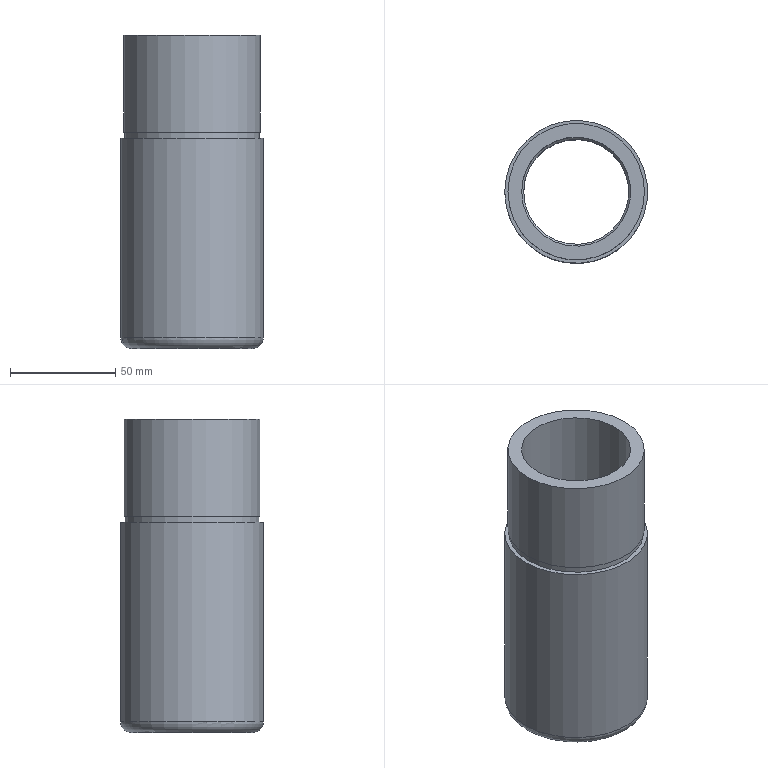Component | NX | OUTER_GUIDE_BUSH | 1 solid | 17 faces | box 68 x 68 x 149 mm | volume 223119 mm3 | cylinder 8 | plane 4 | torus 4 | cone 1 | commonest cylinder face diameters 50 x4 64 x1 68 x1 51.928 x1 64.974 x1
STEP:
#1=CARTESIAN_POINT('',(0.,0.,0.));
#2=DIRECTION('',(0.,0.,1.));
#3=DIRECTION('',(1.,0.,0.));
#4=AXIS2_PLACEMENT_3D('',#1,#2,#3);
#5=CARTESIAN_POINT('',(-322.,-290.,198.));
#6=VERTEX_POINT('',#5);
#7=CARTESIAN_POINT('',(-290.,-290.,198.));
#8=DIRECTION('',(0.,0.,-1.));
#9=DIRECTION('',(-1.,0.0000016,0.));
#10=AXIS2_PLACEMENT_3D('',#7,#8,#9);
#11=CIRCLE('',#10,32.);
#12=CARTESIAN_POINT('',(-257.513,-290.,198.));
#13=DIRECTION('',(0.,0.,1.));
#14=DIRECTION('',(1.,-0.0000016,0.));
#15=AXIS2_PLACEMENT_3D('',#12,#13,#14);
#16=PLANE('',#15);
#17=CARTESIAN_POINT('',(-64.487,-0.));
#18=CARTESIAN_POINT('',(-64.487,55.426));
#19=CARTESIAN_POINT('',(-16.487,27.713));
#20=CARTESIAN_POINT('',(31.513,0.));
#21=CARTESIAN_POINT('',(-16.487,-27.713));
#22=CARTESIAN_POINT('',(-64.487,-55.426));
#23=CARTESIAN_POINT('',(-64.487,-0.));
#24=(BOUNDED_CURVE()B_SPLINE_CURVE(2,(#17,#18,#19,#20,#21,#22,#23),.UNSPECIFIED.,.T.,.F.)B_SPLINE_CURVE_WITH_KNOTS((1,2,2,2,2,1),(-2.094,0.,2.094,4.189,6.283,8.378),.UNSPECIFIED.)CURVE()GEOMETRIC_REPRESENTATION_ITEM()RATIONAL_B_SPLINE_CURVE((1.,0.5,1.,0.5,1.,0.5,1.))REPRESENTATION_ITEM(''));
#25=(GEOMETRIC_REPRESENTATION_CONTEXT(2)PARAMETRIC_REPRESENTATION_CONTEXT()REPRESENTATION_CONTEXT('',''));
#26=DEFINITIONAL_REPRESENTATION('',(#24),#25);
#27=PCURVE('',#16,#26);
#28=CARTESIAN_POINT('',(-290.,-290.,95.));
#29=DIRECTION('',(0.,0.,-1.));
#30=DIRECTION('',(-1.,0.0000016,0.));
#31=AXIS2_PLACEMENT_3D('',#28,#29,#30);
#32=CYLINDRICAL_SURFACE('',#31,32.);
#33=CARTESIAN_POINT('',(0.,-103.));
#34=DIRECTION('',(1.,0.));
#35=VECTOR('',#34,1.);
#36=LINE('',#33,#35);
#37=(GEOMETRIC_REPRESENTATION_CONTEXT(2)PARAMETRIC_REPRESENTATION_CONTEXT()REPRESENTATION_CONTEXT('',''));
#38=DEFINITIONAL_REPRESENTATION('',(#36),#37);
#39=PCURVE('',#32,#38);
#40=SURFACE_CURVE('',#11,(#27,#39),.PCURVE_S1.);
#41=EDGE_CURVE('',#6,#6,#40,.T.);
#42=ORIENTED_EDGE('',*,*,#41,.F.);
#43=EDGE_LOOP('',(#42));
#44=FACE_BOUND('',#43,.T.);
#45=CARTESIAN_POINT('',(-322.487,-290.,198.));
#46=VERTEX_POINT('',#45);
#47=CARTESIAN_POINT('',(-290.,-290.,198.));
#48=DIRECTION('',(0.,0.,-1.));
#49=DIRECTION('',(-1.,0.0000016,0.));
#50=AXIS2_PLACEMENT_3D('',#47,#48,#49);
#51=CIRCLE('',#50,32.487);
#52=CARTESIAN_POINT('',(-64.974,-0.));
#53=CARTESIAN_POINT('',(-64.974,56.269));
#54=CARTESIAN_POINT('',(-16.243,28.134));
#55=CARTESIAN_POINT('',(32.487,0.));
#56=CARTESIAN_POINT('',(-16.243,-28.134));
#57=CARTESIAN_POINT('',(-64.974,-56.269));
#58=CARTESIAN_POINT('',(-64.974,-0.));
#59=(BOUNDED_CURVE()B_SPLINE_CURVE(2,(#52,#53,#54,#55,#56,#57,#58),.UNSPECIFIED.,.T.,.F.)B_SPLINE_CURVE_WITH_KNOTS((1,2,2,2,2,1),(-2.094,0.,2.094,4.189,6.283,8.378),.UNSPECIFIED.)CURVE()GEOMETRIC_REPRESENTATION_ITEM()RATIONAL_B_SPLINE_CURVE((1.,0.5,1.,0.5,1.,0.5,1.))REPRESENTATION_ITEM(''));
#60=(GEOMETRIC_REPRESENTATION_CONTEXT(2)PARAMETRIC_REPRESENTATION_CONTEXT()REPRESENTATION_CONTEXT('',''));
#61=DEFINITIONAL_REPRESENTATION('',(#59),#60);
#62=PCURVE('',#16,#61);
#63=CARTESIAN_POINT('',(-290.,-290.,95.));
#64=DIRECTION('',(0.,0.,-1.));
#65=DIRECTION('',(-1.,0.0000016,0.));
#66=AXIS2_PLACEMENT_3D('',#63,#64,#65);
#67=CYLINDRICAL_SURFACE('',#66,32.487);
#68=CARTESIAN_POINT('',(0.,-103.));
#69=DIRECTION('',(1.,0.));
#70=VECTOR('',#69,1.);
#71=LINE('',#68,#70);
#72=(GEOMETRIC_REPRESENTATION_CONTEXT(2)PARAMETRIC_REPRESENTATION_CONTEXT()REPRESENTATION_CONTEXT('',''));
#73=DEFINITIONAL_REPRESENTATION('',(#71),#72);
#74=PCURVE('',#67,#73);
#75=SURFACE_CURVE('',#51,(#62,#74),.PCURVE_S1.);
#76=EDGE_CURVE('',#46,#46,#75,.T.);
#77=ORIENTED_EDGE('',*,*,#76,.T.);
#78=EDGE_LOOP('',(#77));
#79=FACE_BOUND('',#78,.T.);
#80=ADVANCED_FACE('',(#44,#79),#16,.F.);
#81=CARTESIAN_POINT('',(-322.,-290.,195.));
#82=VERTEX_POINT('',#81);
#83=CARTESIAN_POINT('',(-290.,-290.,195.));
#84=DIRECTION('',(0.,0.,-1.));
#85=DIRECTION('',(-1.,0.0000016,0.));
#86=AXIS2_PLACEMENT_3D('',#83,#84,#85);
#87=CIRCLE('',#86,32.);
#88=CARTESIAN_POINT('',(0.,-100.));
#89=DIRECTION('',(1.,0.));
#90=VECTOR('',#89,1.);
#91=LINE('',#88,#90);
#92=(GEOMETRIC_REPRESENTATION_CONTEXT(2)PARAMETRIC_REPRESENTATION_CONTEXT()REPRESENTATION_CONTEXT('',''));
#93=DEFINITIONAL_REPRESENTATION('',(#91),#92);
#94=PCURVE('',#32,#93);
#95=CARTESIAN_POINT('',(-258.,-290.,195.));
#96=DIRECTION('',(0.,0.,-1.));
#97=DIRECTION('',(-1.,0.0000016,0.));
#98=AXIS2_PLACEMENT_3D('',#95,#96,#97);
#99=PLANE('',#98);
#100=CARTESIAN_POINT('',(32.,-0.));
#101=DIRECTION('',(1.,-0.));
#102=AXIS2_PLACEMENT_2D('',#100,#101);
#103=CIRCLE('',#102,32.);
#104=(GEOMETRIC_REPRESENTATION_CONTEXT(2)PARAMETRIC_REPRESENTATION_CONTEXT()REPRESENTATION_CONTEXT('',''));
#105=DEFINITIONAL_REPRESENTATION('',(#103),#104);
#106=PCURVE('',#99,#105);
#107=SURFACE_CURVE('',#87,(#94,#106),.PCURVE_S1.);
#108=EDGE_CURVE('',#82,#82,#107,.T.);
#109=ORIENTED_EDGE('',*,*,#108,.F.);
#110=CARTESIAN_POINT('',(-322.,-290.,198.));
#111=CARTESIAN_POINT('',(-322.,-290.,195.));
#112=B_SPLINE_CURVE_WITH_KNOTS('',1,(#110,#111),.UNSPECIFIED.,.F.,.F.,(2,2),(-103.,-100.),.PIECEWISE_BEZIER_KNOTS.);
#113=CARTESIAN_POINT('',(0.,0.));
#114=DIRECTION('',(0.,1.));
#115=VECTOR('',#114,1.);
#116=LINE('',#113,#115);
#117=(GEOMETRIC_REPRESENTATION_CONTEXT(2)PARAMETRIC_REPRESENTATION_CONTEXT()REPRESENTATION_CONTEXT('',''));
#118=DEFINITIONAL_REPRESENTATION('',(#116),#117);
#119=PCURVE('',#32,#118);
#120=CARTESIAN_POINT('',(6.283,0.));
#121=DIRECTION('',(0.,1.));
#122=VECTOR('',#121,1.);
#123=LINE('',#120,#122);
#124=(GEOMETRIC_REPRESENTATION_CONTEXT(2)PARAMETRIC_REPRESENTATION_CONTEXT()REPRESENTATION_CONTEXT('',''));
#125=DEFINITIONAL_REPRESENTATION('',(#123),#124);
#126=PCURVE('',#32,#125);
#127=SEAM_CURVE('',#112,(#119,#126),.PCURVE_S1.);
#128=EDGE_CURVE('',#6,#82,#127,.T.);
#129=ORIENTED_EDGE('',*,*,#128,.F.);
#130=ORIENTED_EDGE('',*,*,#41,.T.);
#131=ORIENTED_EDGE('',*,*,#128,.T.);
#132=EDGE_LOOP('',(#109,#129,#130,#131));
#133=FACE_BOUND('',#132,.T.);
#134=ADVANCED_FACE('',(#133),#32,.T.);
#135=CARTESIAN_POINT('',(-324.,-290.,195.));
#136=VERTEX_POINT('',#135);
#137=CARTESIAN_POINT('',(-290.,-290.,195.));
#138=DIRECTION('',(0.,0.,-1.));
#139=DIRECTION('',(-1.,0.0000016,0.));
#140=AXIS2_PLACEMENT_3D('',#137,#138,#139);
#141=CIRCLE('',#140,34.);
#142=CARTESIAN_POINT('',(32.,-0.));
#143=DIRECTION('',(1.,-0.));
#144=AXIS2_PLACEMENT_2D('',#142,#143);
#145=CIRCLE('',#144,34.);
#146=(GEOMETRIC_REPRESENTATION_CONTEXT(2)PARAMETRIC_REPRESENTATION_CONTEXT()REPRESENTATION_CONTEXT('',''));
#147=DEFINITIONAL_REPRESENTATION('',(#145),#146);
#148=PCURVE('',#99,#147);
#149=CARTESIAN_POINT('',(-290.,-290.,95.));
#150=DIRECTION('',(0.,0.,-1.));
#151=DIRECTION('',(-1.,0.0000016,0.));
#152=AXIS2_PLACEMENT_3D('',#149,#150,#151);
#153=CYLINDRICAL_SURFACE('',#152,34.);
#154=CARTESIAN_POINT('',(0.,-100.));
#155=DIRECTION('',(1.,0.));
#156=VECTOR('',#155,1.);
#157=LINE('',#154,#156);
#158=(GEOMETRIC_REPRESENTATION_CONTEXT(2)PARAMETRIC_REPRESENTATION_CONTEXT()REPRESENTATION_CONTEXT('',''));
#159=DEFINITIONAL_REPRESENTATION('',(#157),#158);
#160=PCURVE('',#153,#159);
#161=SURFACE_CURVE('',#141,(#148,#160),.PCURVE_S1.);
#162=EDGE_CURVE('',#136,#136,#161,.T.);
#163=ORIENTED_EDGE('',*,*,#162,.F.);
#164=EDGE_LOOP('',(#163));
#165=FACE_BOUND('',#164,.T.);
#166=ORIENTED_EDGE('',*,*,#108,.T.);
#167=EDGE_LOOP('',(#166));
#168=FACE_BOUND('',#167,.T.);
#169=ADVANCED_FACE('',(#165,#168),#99,.F.);
#170=CARTESIAN_POINT('',(-324.,-290.,100.));
#171=VERTEX_POINT('',#170);
#172=CARTESIAN_POINT('',(-290.,-290.,100.));
#173=DIRECTION('',(0.,0.,-1.));
#174=DIRECTION('',(-1.,0.0000016,0.));
#175=AXIS2_PLACEMENT_3D('',#172,#173,#174);
#176=CIRCLE('',#175,34.);
#177=CARTESIAN_POINT('',(0.,-5.));
#178=DIRECTION('',(1.,0.));
#179=VECTOR('',#178,1.);
#180=LINE('',#177,#179);
#181=(GEOMETRIC_REPRESENTATION_CONTEXT(2)PARAMETRIC_REPRESENTATION_CONTEXT()REPRESENTATION_CONTEXT('',''));
#182=DEFINITIONAL_REPRESENTATION('',(#180),#181);
#183=PCURVE('',#153,#182);
#184=CARTESIAN_POINT('',(-290.,-290.,100.));
#185=DIRECTION('',(0.,0.,-1.));
#186=DIRECTION('',(-1.,0.0000016,0.));
#187=AXIS2_PLACEMENT_3D('',#184,#185,#186);
#188=TOROIDAL_SURFACE('',#187,29.,5.);
#189=CARTESIAN_POINT('',(0.,6.283));
#190=DIRECTION('',(1.,0.));
#191=VECTOR('',#190,1.);
#192=LINE('',#189,#191);
#193=(GEOMETRIC_REPRESENTATION_CONTEXT(2)PARAMETRIC_REPRESENTATION_CONTEXT()REPRESENTATION_CONTEXT('',''));
#194=DEFINITIONAL_REPRESENTATION('',(#192),#193);
#195=PCURVE('',#188,#194);
#196=SURFACE_CURVE('',#176,(#183,#195),.PCURVE_S1.);
#197=EDGE_CURVE('',#171,#171,#196,.T.);
#198=ORIENTED_EDGE('',*,*,#197,.F.);
#199=CARTESIAN_POINT('',(-324.,-290.,195.));
#200=CARTESIAN_POINT('',(-324.,-290.,100.));
#201=B_SPLINE_CURVE_WITH_KNOTS('',1,(#199,#200),.UNSPECIFIED.,.F.,.F.,(2,2),(-100.,-5.),.PIECEWISE_BEZIER_KNOTS.);
#202=CARTESIAN_POINT('',(0.,0.));
#203=DIRECTION('',(0.,1.));
#204=VECTOR('',#203,1.);
#205=LINE('',#202,#204);
#206=(GEOMETRIC_REPRESENTATION_CONTEXT(2)PARAMETRIC_REPRESENTATION_CONTEXT()REPRESENTATION_CONTEXT('',''));
#207=DEFINITIONAL_REPRESENTATION('',(#205),#206);
#208=PCURVE('',#153,#207);
#209=CARTESIAN_POINT('',(6.283,0.));
#210=DIRECTION('',(0.,1.));
#211=VECTOR('',#210,1.);
#212=LINE('',#209,#211);
#213=(GEOMETRIC_REPRESENTATION_CONTEXT(2)PARAMETRIC_REPRESENTATION_CONTEXT()REPRESENTATION_CONTEXT('',''));
#214=DEFINITIONAL_REPRESENTATION('',(#212),#213);
#215=PCURVE('',#153,#214);
#216=SEAM_CURVE('',#201,(#208,#215),.PCURVE_S1.);
#217=EDGE_CURVE('',#136,#171,#216,.T.);
#218=ORIENTED_EDGE('',*,*,#217,.F.);
#219=ORIENTED_EDGE('',*,*,#162,.T.);
#220=ORIENTED_EDGE('',*,*,#217,.T.);
#221=EDGE_LOOP('',(#198,#218,#219,#220));
#222=FACE_BOUND('',#221,.T.);
#223=ADVANCED_FACE('',(#222),#153,.T.);
#224=CARTESIAN_POINT('',(-319.,-290.,95.));
#225=VERTEX_POINT('',#224);
#226=CARTESIAN_POINT('',(-290.,-290.,95.));
#227=DIRECTION('',(0.,0.,-1.));
#228=DIRECTION('',(-1.,0.0000016,0.));
#229=AXIS2_PLACEMENT_3D('',#226,#227,#228);
#230=CIRCLE('',#229,29.);
#231=CARTESIAN_POINT('',(0.,7.854));
#232=DIRECTION('',(1.,0.));
#233=VECTOR('',#232,1.);
#234=LINE('',#231,#233);
#235=(GEOMETRIC_REPRESENTATION_CONTEXT(2)PARAMETRIC_REPRESENTATION_CONTEXT()REPRESENTATION_CONTEXT('',''));
#236=DEFINITIONAL_REPRESENTATION('',(#234),#235);
#237=PCURVE('',#188,#236);
#238=CARTESIAN_POINT('',(-261.,-290.,95.));
#239=DIRECTION('',(0.,0.,1.));
#240=DIRECTION('',(1.,-0.0000016,0.));
#241=AXIS2_PLACEMENT_3D('',#238,#239,#240);
#242=PLANE('',#241);
#243=CARTESIAN_POINT('',(-58.,0.));
#244=CARTESIAN_POINT('',(-58.,50.229));
#245=CARTESIAN_POINT('',(-14.5,25.115));
#246=CARTESIAN_POINT('',(29.,0.));
#247=CARTESIAN_POINT('',(-14.5,-25.115));
#248=CARTESIAN_POINT('',(-58.,-50.229));
#249=CARTESIAN_POINT('',(-58.,0.));
#250=(BOUNDED_CURVE()B_SPLINE_CURVE(2,(#243,#244,#245,#246,#247,#248,#249),.UNSPECIFIED.,.T.,.F.)B_SPLINE_CURVE_WITH_KNOTS((1,2,2,2,2,1),(-2.094,0.,2.094,4.189,6.283,8.378),.UNSPECIFIED.)CURVE()GEOMETRIC_REPRESENTATION_ITEM()RATIONAL_B_SPLINE_CURVE((1.,0.5,1.,0.5,1.,0.5,1.))REPRESENTATION_ITEM(''));
#251=(GEOMETRIC_REPRESENTATION_CONTEXT(2)PARAMETRIC_REPRESENTATION_CONTEXT()REPRESENTATION_CONTEXT('',''));
#252=DEFINITIONAL_REPRESENTATION('',(#250),#251);
#253=PCURVE('',#242,#252);
#254=SURFACE_CURVE('',#230,(#237,#253),.PCURVE_S1.);
#255=EDGE_CURVE('',#225,#225,#254,.T.);
#256=ORIENTED_EDGE('',*,*,#255,.F.);
#257=CARTESIAN_POINT('',(-324.,-290.,100.));
#258=CARTESIAN_POINT('',(-324.,-290.,98.663));
#259=CARTESIAN_POINT('',(-323.575,-290.,97.361));
#260=CARTESIAN_POINT('',(-322.76,-290.,96.24));
#261=CARTESIAN_POINT('',(-321.639,-290.,95.425));
#262=CARTESIAN_POINT('',(-320.337,-290.,95.));
#263=CARTESIAN_POINT('',(-319.,-290.,95.));
#264=(BOUNDED_CURVE()B_SPLINE_CURVE(6,(#257,#258,#259,#260,#261,#262,#263),.UNSPECIFIED.,.F.,.F.)B_SPLINE_CURVE_WITH_KNOTS((7,7),(0.,1.571),.PIECEWISE_BEZIER_KNOTS.)CURVE()GEOMETRIC_REPRESENTATION_ITEM()RATIONAL_B_SPLINE_CURVE((1.031,1.01,0.9979,0.994,0.9979,1.01,1.031))REPRESENTATION_ITEM(''));
#265=CARTESIAN_POINT('',(0.,6.283));
#266=DIRECTION('',(0.,1.));
#267=VECTOR('',#266,1.);
#268=LINE('',#265,#267);
#269=(GEOMETRIC_REPRESENTATION_CONTEXT(2)PARAMETRIC_REPRESENTATION_CONTEXT()REPRESENTATION_CONTEXT('',''));
#270=DEFINITIONAL_REPRESENTATION('',(#268),#269);
#271=PCURVE('',#188,#270);
#272=CARTESIAN_POINT('',(6.283,6.283));
#273=DIRECTION('',(0.,1.));
#274=VECTOR('',#273,1.);
#275=LINE('',#272,#274);
#276=(GEOMETRIC_REPRESENTATION_CONTEXT(2)PARAMETRIC_REPRESENTATION_CONTEXT()REPRESENTATION_CONTEXT('',''));
#277=DEFINITIONAL_REPRESENTATION('',(#275),#276);
#278=PCURVE('',#188,#277);
#279=SEAM_CURVE('',#264,(#271,#278),.PCURVE_S1.);
#280=EDGE_CURVE('',#171,#225,#279,.T.);
#281=ORIENTED_EDGE('',*,*,#280,.F.);
#282=ORIENTED_EDGE('',*,*,#197,.T.);
#283=ORIENTED_EDGE('',*,*,#280,.T.);
#284=EDGE_LOOP('',(#256,#281,#282,#283));
#285=FACE_BOUND('',#284,.T.);
#286=ADVANCED_FACE('',(#285),#188,.T.);
#287=CARTESIAN_POINT('',(-315.,-290.,95.));
#288=VERTEX_POINT('',#287);
#289=CARTESIAN_POINT('',(-290.,-290.,95.));
#290=DIRECTION('',(0.,0.,-1.));
#291=DIRECTION('',(-1.,0.0000016,0.));
#292=AXIS2_PLACEMENT_3D('',#289,#290,#291);
#293=CIRCLE('',#292,25.);
#294=CARTESIAN_POINT('',(-54.,0.));
#295=CARTESIAN_POINT('',(-54.,43.301));
#296=CARTESIAN_POINT('',(-16.5,21.651));
#297=CARTESIAN_POINT('',(21.,0.));
#298=CARTESIAN_POINT('',(-16.5,-21.651));
#299=CARTESIAN_POINT('',(-54.,-43.301));
#300=CARTESIAN_POINT('',(-54.,0.));
#301=(BOUNDED_CURVE()B_SPLINE_CURVE(2,(#294,#295,#296,#297,#298,#299,#300),.UNSPECIFIED.,.T.,.F.)B_SPLINE_CURVE_WITH_KNOTS((1,2,2,2,2,1),(-2.094,0.,2.094,4.189,6.283,8.378),.UNSPECIFIED.)CURVE()GEOMETRIC_REPRESENTATION_ITEM()RATIONAL_B_SPLINE_CURVE((1.,0.5,1.,0.5,1.,0.5,1.))REPRESENTATION_ITEM(''));
#302=(GEOMETRIC_REPRESENTATION_CONTEXT(2)PARAMETRIC_REPRESENTATION_CONTEXT()REPRESENTATION_CONTEXT('',''));
#303=DEFINITIONAL_REPRESENTATION('',(#301),#302);
#304=PCURVE('',#242,#303);
#305=CARTESIAN_POINT('',(-290.,-290.,95.));
#306=DIRECTION('',(0.,0.,-1.));
#307=DIRECTION('',(-1.,0.0000016,0.));
#308=AXIS2_PLACEMENT_3D('',#305,#306,#307);
#309=CYLINDRICAL_SURFACE('',#308,25.);
#310=CARTESIAN_POINT('',(0.,0.));
#311=DIRECTION('',(1.,0.));
#312=VECTOR('',#311,1.);
#313=LINE('',#310,#312);
#314=(GEOMETRIC_REPRESENTATION_CONTEXT(2)PARAMETRIC_REPRESENTATION_CONTEXT()REPRESENTATION_CONTEXT('',''));
#315=DEFINITIONAL_REPRESENTATION('',(#313),#314);
#316=PCURVE('',#309,#315);
#317=SURFACE_CURVE('',#293,(#304,#316),.PCURVE_S1.);
#318=EDGE_CURVE('',#288,#288,#317,.T.);
#319=ORIENTED_EDGE('',*,*,#318,.F.);
#320=EDGE_LOOP('',(#319));
#321=FACE_BOUND('',#320,.T.);
#322=ORIENTED_EDGE('',*,*,#255,.T.);
#323=EDGE_LOOP('',(#322));
#324=FACE_BOUND('',#323,.T.);
#325=ADVANCED_FACE('',(#321,#324),#242,.F.);
#326=CARTESIAN_POINT('',(-315.,-290.,105.538));
#327=VERTEX_POINT('',#326);
#328=CARTESIAN_POINT('',(-290.,-290.,105.538));
#329=DIRECTION('',(0.,0.,-1.));
#330=DIRECTION('',(-1.,0.0000016,0.));
#331=AXIS2_PLACEMENT_3D('',#328,#329,#330);
#332=CIRCLE('',#331,25.);
#333=CARTESIAN_POINT('',(0.,-10.538));
#334=DIRECTION('',(1.,0.));
#335=VECTOR('',#334,1.);
#336=LINE('',#333,#335);
#337=(GEOMETRIC_REPRESENTATION_CONTEXT(2)PARAMETRIC_REPRESENTATION_CONTEXT()REPRESENTATION_CONTEXT('',''));
#338=DEFINITIONAL_REPRESENTATION('',(#336),#337);
#339=PCURVE('',#309,#338);
#340=CARTESIAN_POINT('',(-290.,-290.,106.538));
#341=DIRECTION('',(0.,0.,-1.));
#342=DIRECTION('',(-1.,0.0000016,0.));
#343=AXIS2_PLACEMENT_3D('',#340,#341,#342);
#344=TOROIDAL_SURFACE('',#343,25.,1.);
#345=CARTESIAN_POINT('',(0.,7.854));
#346=DIRECTION('',(1.,0.));
#347=VECTOR('',#346,1.);
#348=LINE('',#345,#347);
#349=(GEOMETRIC_REPRESENTATION_CONTEXT(2)PARAMETRIC_REPRESENTATION_CONTEXT()REPRESENTATION_CONTEXT('',''));
#350=DEFINITIONAL_REPRESENTATION('',(#348),#349);
#351=PCURVE('',#344,#350);
#352=SURFACE_CURVE('',#332,(#339,#351),.PCURVE_S1.);
#353=EDGE_CURVE('',#327,#327,#352,.T.);
#354=ORIENTED_EDGE('',*,*,#353,.T.);
#355=CARTESIAN_POINT('',(-315.,-290.,105.538));
#356=CARTESIAN_POINT('',(-315.,-290.,95.));
#357=B_SPLINE_CURVE_WITH_KNOTS('',1,(#355,#356),.UNSPECIFIED.,.F.,.F.,(2,2),(-10.538,0.),.PIECEWISE_BEZIER_KNOTS.);
#358=CARTESIAN_POINT('',(6.283,0.));
#359=DIRECTION('',(0.,1.));
#360=VECTOR('',#359,1.);
#361=LINE('',#358,#360);
#362=(GEOMETRIC_REPRESENTATION_CONTEXT(2)PARAMETRIC_REPRESENTATION_CONTEXT()REPRESENTATION_CONTEXT('',''));
#363=DEFINITIONAL_REPRESENTATION('',(#361),#362);
#364=PCURVE('',#309,#363);
#365=CARTESIAN_POINT('',(0.,0.));
#366=DIRECTION('',(0.,1.));
#367=VECTOR('',#366,1.);
#368=LINE('',#365,#367);
#369=(GEOMETRIC_REPRESENTATION_CONTEXT(2)PARAMETRIC_REPRESENTATION_CONTEXT()REPRESENTATION_CONTEXT('',''));
#370=DEFINITIONAL_REPRESENTATION('',(#368),#369);
#371=PCURVE('',#309,#370);
#372=SEAM_CURVE('',#357,(#364,#371),.PCURVE_S1.);
#373=EDGE_CURVE('',#327,#288,#372,.T.);
#374=ORIENTED_EDGE('',*,*,#373,.T.);
#375=ORIENTED_EDGE('',*,*,#318,.F.);
#376=ORIENTED_EDGE('',*,*,#373,.F.);
#377=EDGE_LOOP('',(#354,#374,#375,#376));
#378=FACE_BOUND('',#377,.F.);
#379=ADVANCED_FACE('',(#378),#309,.F.);
#380=CARTESIAN_POINT('',(-315.,-290.,107.538));
#381=VERTEX_POINT('',#380);
#382=CARTESIAN_POINT('',(-290.,-290.,107.538));
#383=DIRECTION('',(0.,0.,-1.));
#384=DIRECTION('',(-1.,0.0000016,0.));
#385=AXIS2_PLACEMENT_3D('',#382,#383,#384);
#386=CIRCLE('',#385,25.);
#387=CARTESIAN_POINT('',(0.,4.712));
#388=DIRECTION('',(1.,0.));
#389=VECTOR('',#388,1.);
#390=LINE('',#387,#389);
#391=(GEOMETRIC_REPRESENTATION_CONTEXT(2)PARAMETRIC_REPRESENTATION_CONTEXT()REPRESENTATION_CONTEXT('',''));
#392=DEFINITIONAL_REPRESENTATION('',(#390),#391);
#393=PCURVE('',#344,#392);
#394=CARTESIAN_POINT('',(-290.,-290.,95.));
#395=DIRECTION('',(0.,0.,-1.));
#396=DIRECTION('',(-1.,0.0000016,0.));
#397=AXIS2_PLACEMENT_3D('',#394,#395,#396);
#398=CYLINDRICAL_SURFACE('',#397,25.);
#399=CARTESIAN_POINT('',(0.,-12.538));
#400=DIRECTION('',(1.,0.));
#401=VECTOR('',#400,1.);
#402=LINE('',#399,#401);
#403=(GEOMETRIC_REPRESENTATION_CONTEXT(2)PARAMETRIC_REPRESENTATION_CONTEXT()REPRESENTATION_CONTEXT('',''));
#404=DEFINITIONAL_REPRESENTATION('',(#402),#403);
#405=PCURVE('',#398,#404);
#406=SURFACE_CURVE('',#386,(#393,#405),.PCURVE_S1.);
#407=EDGE_CURVE('',#381,#381,#406,.T.);
#408=ORIENTED_EDGE('',*,*,#407,.T.);
#409=CARTESIAN_POINT('',(-315.,-290.,107.538));
#410=CARTESIAN_POINT('',(-315.393,-290.,107.538));
#411=CARTESIAN_POINT('',(-315.785,-290.,107.362));
#412=CARTESIAN_POINT('',(-316.086,-290.,107.01));
#413=CARTESIAN_POINT('',(-316.202,-290.,106.538));
#414=CARTESIAN_POINT('',(-316.086,-290.,106.067));
#415=CARTESIAN_POINT('',(-315.785,-290.,105.715));
#416=CARTESIAN_POINT('',(-315.393,-290.,105.538));
#417=CARTESIAN_POINT('',(-315.,-290.,105.538));
#418=B_SPLINE_CURVE_WITH_KNOTS('',8,(#409,#410,#411,#412,#413,#414,#415,#416,#417),.UNSPECIFIED.,.F.,.F.,(9,9),(4.712,7.854),.PIECEWISE_BEZIER_KNOTS.);
#419=CARTESIAN_POINT('',(6.283,0.));
#420=DIRECTION('',(0.,1.));
#421=VECTOR('',#420,1.);
#422=LINE('',#419,#421);
#423=(GEOMETRIC_REPRESENTATION_CONTEXT(2)PARAMETRIC_REPRESENTATION_CONTEXT()REPRESENTATION_CONTEXT('',''));
#424=DEFINITIONAL_REPRESENTATION('',(#422),#423);
#425=PCURVE('',#344,#424);
#426=CARTESIAN_POINT('',(0.,0.));
#427=DIRECTION('',(0.,1.));
#428=VECTOR('',#427,1.);
#429=LINE('',#426,#428);
#430=(GEOMETRIC_REPRESENTATION_CONTEXT(2)PARAMETRIC_REPRESENTATION_CONTEXT()REPRESENTATION_CONTEXT('',''));
#431=DEFINITIONAL_REPRESENTATION('',(#429),#430);
#432=PCURVE('',#344,#431);
#433=SEAM_CURVE('',#418,(#425,#432),.PCURVE_S1.);
#434=EDGE_CURVE('',#381,#327,#433,.T.);
#435=ORIENTED_EDGE('',*,*,#434,.T.);
#436=ORIENTED_EDGE('',*,*,#353,.F.);
#437=ORIENTED_EDGE('',*,*,#434,.F.);
#438=EDGE_LOOP('',(#408,#435,#436,#437));
#439=FACE_BOUND('',#438,.F.);
#440=ADVANCED_FACE('',(#439),#344,.F.);
#441=CARTESIAN_POINT('',(-315.,-290.,135.538));
#442=VERTEX_POINT('',#441);
#443=CARTESIAN_POINT('',(-290.,-290.,135.538));
#444=DIRECTION('',(0.,0.,-1.));
#445=DIRECTION('',(-1.,0.0000016,0.));
#446=AXIS2_PLACEMENT_3D('',#443,#444,#445);
#447=CIRCLE('',#446,25.);
#448=CARTESIAN_POINT('',(0.,-40.538));
#449=DIRECTION('',(1.,0.));
#450=VECTOR('',#449,1.);
#451=LINE('',#448,#450);
#452=(GEOMETRIC_REPRESENTATION_CONTEXT(2)PARAMETRIC_REPRESENTATION_CONTEXT()REPRESENTATION_CONTEXT('',''));
#453=DEFINITIONAL_REPRESENTATION('',(#451),#452);
#454=PCURVE('',#398,#453);
#455=CARTESIAN_POINT('',(-290.,-290.,136.538));
#456=DIRECTION('',(0.,0.,-1.));
#457=DIRECTION('',(-1.,0.0000016,0.));
#458=AXIS2_PLACEMENT_3D('',#455,#456,#457);
#459=TOROIDAL_SURFACE('',#458,25.,1.);
#460=CARTESIAN_POINT('',(0.,7.854));
#461=DIRECTION('',(1.,0.));
#462=VECTOR('',#461,1.);
#463=LINE('',#460,#462);
#464=(GEOMETRIC_REPRESENTATION_CONTEXT(2)PARAMETRIC_REPRESENTATION_CONTEXT()REPRESENTATION_CONTEXT('',''));
#465=DEFINITIONAL_REPRESENTATION('',(#463),#464);
#466=PCURVE('',#459,#465);
#467=SURFACE_CURVE('',#447,(#454,#466),.PCURVE_S1.);
#468=EDGE_CURVE('',#442,#442,#467,.T.);
#469=ORIENTED_EDGE('',*,*,#468,.T.);
#470=CARTESIAN_POINT('',(-315.,-290.,135.538));
#471=CARTESIAN_POINT('',(-315.,-290.,107.538));
#472=B_SPLINE_CURVE_WITH_KNOTS('',1,(#470,#471),.UNSPECIFIED.,.F.,.F.,(2,2),(-40.538,-12.538),.PIECEWISE_BEZIER_KNOTS.);
#473=CARTESIAN_POINT('',(6.283,0.));
#474=DIRECTION('',(0.,1.));
#475=VECTOR('',#474,1.);
#476=LINE('',#473,#475);
#477=(GEOMETRIC_REPRESENTATION_CONTEXT(2)PARAMETRIC_REPRESENTATION_CONTEXT()REPRESENTATION_CONTEXT('',''));
#478=DEFINITIONAL_REPRESENTATION('',(#476),#477);
#479=PCURVE('',#398,#478);
#480=CARTESIAN_POINT('',(0.,0.));
#481=DIRECTION('',(0.,1.));
#482=VECTOR('',#481,1.);
#483=LINE('',#480,#482);
#484=(GEOMETRIC_REPRESENTATION_CONTEXT(2)PARAMETRIC_REPRESENTATION_CONTEXT()REPRESENTATION_CONTEXT('',''));
#485=DEFINITIONAL_REPRESENTATION('',(#483),#484);
#486=PCURVE('',#398,#485);
#487=SEAM_CURVE('',#472,(#479,#486),.PCURVE_S1.);
#488=EDGE_CURVE('',#442,#381,#487,.T.);
#489=ORIENTED_EDGE('',*,*,#488,.T.);
#490=ORIENTED_EDGE('',*,*,#407,.F.);
#491=ORIENTED_EDGE('',*,*,#488,.F.);
#492=EDGE_LOOP('',(#469,#489,#490,#491));
#493=FACE_BOUND('',#492,.F.);
#494=ADVANCED_FACE('',(#493),#398,.F.);
#495=CARTESIAN_POINT('',(-315.,-290.,137.538));
#496=VERTEX_POINT('',#495);
#497=CARTESIAN_POINT('',(-290.,-290.,137.538));
#498=DIRECTION('',(0.,0.,-1.));
#499=DIRECTION('',(-1.,0.0000016,0.));
#500=AXIS2_PLACEMENT_3D('',#497,#498,#499);
#501=CIRCLE('',#500,25.);
#502=CARTESIAN_POINT('',(0.,4.712));
#503=DIRECTION('',(1.,0.));
#504=VECTOR('',#503,1.);
#505=LINE('',#502,#504);
#506=(GEOMETRIC_REPRESENTATION_CONTEXT(2)PARAMETRIC_REPRESENTATION_CONTEXT()REPRESENTATION_CONTEXT('',''));
#507=DEFINITIONAL_REPRESENTATION('',(#505),#506);
#508=PCURVE('',#459,#507);
#509=CARTESIAN_POINT('',(-290.,-290.,95.));
#510=DIRECTION('',(0.,0.,-1.));
#511=DIRECTION('',(-1.,0.0000016,0.));
#512=AXIS2_PLACEMENT_3D('',#509,#510,#511);
#513=CYLINDRICAL_SURFACE('',#512,25.);
#514=CARTESIAN_POINT('',(0.,-42.538));
#515=DIRECTION('',(1.,0.));
#516=VECTOR('',#515,1.);
#517=LINE('',#514,#516);
#518=(GEOMETRIC_REPRESENTATION_CONTEXT(2)PARAMETRIC_REPRESENTATION_CONTEXT()REPRESENTATION_CONTEXT('',''));
#519=DEFINITIONAL_REPRESENTATION('',(#517),#518);
#520=PCURVE('',#513,#519);
#521=SURFACE_CURVE('',#501,(#508,#520),.PCURVE_S1.);
#522=EDGE_CURVE('',#496,#496,#521,.T.);
#523=ORIENTED_EDGE('',*,*,#522,.T.);
#524=CARTESIAN_POINT('',(-315.,-290.,137.538));
#525=CARTESIAN_POINT('',(-315.393,-290.,137.538));
#526=CARTESIAN_POINT('',(-315.785,-290.,137.362));
#527=CARTESIAN_POINT('',(-316.086,-290.,137.01));
#528=CARTESIAN_POINT('',(-316.202,-290.,136.538));
#529=CARTESIAN_POINT('',(-316.086,-290.,136.067));
#530=CARTESIAN_POINT('',(-315.785,-290.,135.715));
#531=CARTESIAN_POINT('',(-315.393,-290.,135.538));
#532=CARTESIAN_POINT('',(-315.,-290.,135.538));
#533=B_SPLINE_CURVE_WITH_KNOTS('',8,(#524,#525,#526,#527,#528,#529,#530,#531,#532),.UNSPECIFIED.,.F.,.F.,(9,9),(4.712,7.854),.PIECEWISE_BEZIER_KNOTS.);
#534=CARTESIAN_POINT('',(6.283,0.));
#535=DIRECTION('',(0.,1.));
#536=VECTOR('',#535,1.);
#537=LINE('',#534,#536);
#538=(GEOMETRIC_REPRESENTATION_CONTEXT(2)PARAMETRIC_REPRESENTATION_CONTEXT()REPRESENTATION_CONTEXT('',''));
#539=DEFINITIONAL_REPRESENTATION('',(#537),#538);
#540=PCURVE('',#459,#539);
#541=CARTESIAN_POINT('',(0.,0.));
#542=DIRECTION('',(0.,1.));
#543=VECTOR('',#542,1.);
#544=LINE('',#541,#543);
#545=(GEOMETRIC_REPRESENTATION_CONTEXT(2)PARAMETRIC_REPRESENTATION_CONTEXT()REPRESENTATION_CONTEXT('',''));
#546=DEFINITIONAL_REPRESENTATION('',(#544),#545);
#547=PCURVE('',#459,#546);
#548=SEAM_CURVE('',#533,(#540,#547),.PCURVE_S1.);
#549=EDGE_CURVE('',#496,#442,#548,.T.);
#550=ORIENTED_EDGE('',*,*,#549,.T.);
#551=ORIENTED_EDGE('',*,*,#468,.F.);
#552=ORIENTED_EDGE('',*,*,#549,.F.);
#553=EDGE_LOOP('',(#523,#550,#551,#552));
#554=FACE_BOUND('',#553,.F.);
#555=ADVANCED_FACE('',(#554),#459,.F.);
#556=CARTESIAN_POINT('',(-315.,-290.,165.538));
#557=VERTEX_POINT('',#556);
#558=CARTESIAN_POINT('',(-290.,-290.,165.538));
#559=DIRECTION('',(0.,0.,-1.));
#560=DIRECTION('',(-1.,0.0000016,0.));
#561=AXIS2_PLACEMENT_3D('',#558,#559,#560);
#562=CIRCLE('',#561,25.);
#563=CARTESIAN_POINT('',(0.,-70.538));
#564=DIRECTION('',(1.,0.));
#565=VECTOR('',#564,1.);
#566=LINE('',#563,#565);
#567=(GEOMETRIC_REPRESENTATION_CONTEXT(2)PARAMETRIC_REPRESENTATION_CONTEXT()REPRESENTATION_CONTEXT('',''));
#568=DEFINITIONAL_REPRESENTATION('',(#566),#567);
#569=PCURVE('',#513,#568);
#570=CARTESIAN_POINT('',(-290.,-290.,166.538));
#571=DIRECTION('',(0.,0.,-1.));
#572=DIRECTION('',(-1.,0.0000016,0.));
#573=AXIS2_PLACEMENT_3D('',#570,#571,#572);
#574=TOROIDAL_SURFACE('',#573,25.,1.);
#575=CARTESIAN_POINT('',(0.,7.854));
#576=DIRECTION('',(1.,0.));
#577=VECTOR('',#576,1.);
#578=LINE('',#575,#577);
#579=(GEOMETRIC_REPRESENTATION_CONTEXT(2)PARAMETRIC_REPRESENTATION_CONTEXT()REPRESENTATION_CONTEXT('',''));
#580=DEFINITIONAL_REPRESENTATION('',(#578),#579);
#581=PCURVE('',#574,#580);
#582=SURFACE_CURVE('',#562,(#569,#581),.PCURVE_S1.);
#583=EDGE_CURVE('',#557,#557,#582,.T.);
#584=ORIENTED_EDGE('',*,*,#583,.T.);
#585=CARTESIAN_POINT('',(-315.,-290.,165.538));
#586=CARTESIAN_POINT('',(-315.,-290.,137.538));
#587=B_SPLINE_CURVE_WITH_KNOTS('',1,(#585,#586),.UNSPECIFIED.,.F.,.F.,(2,2),(-70.538,-42.538),.PIECEWISE_BEZIER_KNOTS.);
#588=CARTESIAN_POINT('',(6.283,0.));
#589=DIRECTION('',(0.,1.));
#590=VECTOR('',#589,1.);
#591=LINE('',#588,#590);
#592=(GEOMETRIC_REPRESENTATION_CONTEXT(2)PARAMETRIC_REPRESENTATION_CONTEXT()REPRESENTATION_CONTEXT('',''));
#593=DEFINITIONAL_REPRESENTATION('',(#591),#592);
#594=PCURVE('',#513,#593);
#595=CARTESIAN_POINT('',(0.,0.));
#596=DIRECTION('',(0.,1.));
#597=VECTOR('',#596,1.);
#598=LINE('',#595,#597);
#599=(GEOMETRIC_REPRESENTATION_CONTEXT(2)PARAMETRIC_REPRESENTATION_CONTEXT()REPRESENTATION_CONTEXT('',''));
#600=DEFINITIONAL_REPRESENTATION('',(#598),#599);
#601=PCURVE('',#513,#600);
#602=SEAM_CURVE('',#587,(#594,#601),.PCURVE_S1.);
#603=EDGE_CURVE('',#557,#496,#602,.T.);
#604=ORIENTED_EDGE('',*,*,#603,.T.);
#605=ORIENTED_EDGE('',*,*,#522,.F.);
#606=ORIENTED_EDGE('',*,*,#603,.F.);
#607=EDGE_LOOP('',(#584,#604,#605,#606));
#608=FACE_BOUND('',#607,.F.);
#609=ADVANCED_FACE('',(#608),#513,.F.);
#610=CARTESIAN_POINT('',(-315.,-290.,167.538));
#611=VERTEX_POINT('',#610);
#612=CARTESIAN_POINT('',(-290.,-290.,167.538));
#613=DIRECTION('',(0.,0.,-1.));
#614=DIRECTION('',(-1.,0.0000016,0.));
#615=AXIS2_PLACEMENT_3D('',#612,#613,#614);
#616=CIRCLE('',#615,25.);
#617=CARTESIAN_POINT('',(0.,4.712));
#618=DIRECTION('',(1.,0.));
#619=VECTOR('',#618,1.);
#620=LINE('',#617,#619);
#621=(GEOMETRIC_REPRESENTATION_CONTEXT(2)PARAMETRIC_REPRESENTATION_CONTEXT()REPRESENTATION_CONTEXT('',''));
#622=DEFINITIONAL_REPRESENTATION('',(#620),#621);
#623=PCURVE('',#574,#622);
#624=CARTESIAN_POINT('',(-290.,-290.,95.));
#625=DIRECTION('',(0.,0.,-1.));
#626=DIRECTION('',(-1.,0.0000016,0.));
#627=AXIS2_PLACEMENT_3D('',#624,#625,#626);
#628=CYLINDRICAL_SURFACE('',#627,25.);
#629=CARTESIAN_POINT('',(0.,-72.538));
#630=DIRECTION('',(1.,0.));
#631=VECTOR('',#630,1.);
#632=LINE('',#629,#631);
#633=(GEOMETRIC_REPRESENTATION_CONTEXT(2)PARAMETRIC_REPRESENTATION_CONTEXT()REPRESENTATION_CONTEXT('',''));
#634=DEFINITIONAL_REPRESENTATION('',(#632),#633);
#635=PCURVE('',#628,#634);
#636=SURFACE_CURVE('',#616,(#623,#635),.PCURVE_S1.);
#637=EDGE_CURVE('',#611,#611,#636,.T.);
#638=ORIENTED_EDGE('',*,*,#637,.T.);
#639=CARTESIAN_POINT('',(-315.,-290.,167.538));
#640=CARTESIAN_POINT('',(-315.393,-290.,167.538));
#641=CARTESIAN_POINT('',(-315.785,-290.,167.362));
#642=CARTESIAN_POINT('',(-316.086,-290.,167.01));
#643=CARTESIAN_POINT('',(-316.202,-290.,166.538));
#644=CARTESIAN_POINT('',(-316.086,-290.,166.067));
#645=CARTESIAN_POINT('',(-315.785,-290.,165.715));
#646=CARTESIAN_POINT('',(-315.393,-290.,165.538));
#647=CARTESIAN_POINT('',(-315.,-290.,165.538));
#648=B_SPLINE_CURVE_WITH_KNOTS('',8,(#639,#640,#641,#642,#643,#644,#645,#646,#647),.UNSPECIFIED.,.F.,.F.,(9,9),(4.712,7.854),.PIECEWISE_BEZIER_KNOTS.);
#649=CARTESIAN_POINT('',(6.283,0.));
#650=DIRECTION('',(0.,1.));
#651=VECTOR('',#650,1.);
#652=LINE('',#649,#651);
#653=(GEOMETRIC_REPRESENTATION_CONTEXT(2)PARAMETRIC_REPRESENTATION_CONTEXT()REPRESENTATION_CONTEXT('',''));
#654=DEFINITIONAL_REPRESENTATION('',(#652),#653);
#655=PCURVE('',#574,#654);
#656=CARTESIAN_POINT('',(0.,0.));
#657=DIRECTION('',(0.,1.));
#658=VECTOR('',#657,1.);
#659=LINE('',#656,#658);
#660=(GEOMETRIC_REPRESENTATION_CONTEXT(2)PARAMETRIC_REPRESENTATION_CONTEXT()REPRESENTATION_CONTEXT('',''));
#661=DEFINITIONAL_REPRESENTATION('',(#659),#660);
#662=PCURVE('',#574,#661);
#663=SEAM_CURVE('',#648,(#655,#662),.PCURVE_S1.);
#664=EDGE_CURVE('',#611,#557,#663,.T.);
#665=ORIENTED_EDGE('',*,*,#664,.T.);
#666=ORIENTED_EDGE('',*,*,#583,.F.);
#667=ORIENTED_EDGE('',*,*,#664,.F.);
#668=EDGE_LOOP('',(#638,#665,#666,#667));
#669=FACE_BOUND('',#668,.F.);
#670=ADVANCED_FACE('',(#669),#574,.F.);
#671=CARTESIAN_POINT('',(-315.,-290.,193.));
#672=VERTEX_POINT('',#671);
#673=CARTESIAN_POINT('',(-290.,-290.,193.));
#674=DIRECTION('',(0.,0.,-1.));
#675=DIRECTION('',(-1.,0.0000016,0.));
#676=AXIS2_PLACEMENT_3D('',#673,#674,#675);
#677=CIRCLE('',#676,25.);
#678=CARTESIAN_POINT('',(0.,-98.));
#679=DIRECTION('',(1.,0.));
#680=VECTOR('',#679,1.);
#681=LINE('',#678,#680);
#682=(GEOMETRIC_REPRESENTATION_CONTEXT(2)PARAMETRIC_REPRESENTATION_CONTEXT()REPRESENTATION_CONTEXT('',''));
#683=DEFINITIONAL_REPRESENTATION('',(#681),#682);
#684=PCURVE('',#628,#683);
#685=CARTESIAN_POINT('',(-290.,-290.,193.));
#686=DIRECTION('',(0.,0.,1.));
#687=DIRECTION('',(1.,-0.0000016,0.));
#688=AXIS2_PLACEMENT_3D('',#685,#686,#687);
#689=CONICAL_SURFACE('',#688,25.,0.7672);
#690=CARTESIAN_POINT('',(9.425,-0.));
#691=DIRECTION('',(-1.,0.));
#692=VECTOR('',#691,1.);
#693=LINE('',#690,#692);
#694=(GEOMETRIC_REPRESENTATION_CONTEXT(2)PARAMETRIC_REPRESENTATION_CONTEXT()REPRESENTATION_CONTEXT('',''));
#695=DEFINITIONAL_REPRESENTATION('',(#693),#694);
#696=PCURVE('',#689,#695);
#697=SURFACE_CURVE('',#677,(#684,#696),.PCURVE_S1.);
#698=EDGE_CURVE('',#672,#672,#697,.T.);
#699=ORIENTED_EDGE('',*,*,#698,.T.);
#700=CARTESIAN_POINT('',(-315.,-290.,193.));
#701=CARTESIAN_POINT('',(-315.,-290.,167.538));
#702=B_SPLINE_CURVE_WITH_KNOTS('',1,(#700,#701),.UNSPECIFIED.,.F.,.F.,(2,2),(-98.,-72.538),.PIECEWISE_BEZIER_KNOTS.);
#703=CARTESIAN_POINT('',(6.283,0.));
#704=DIRECTION('',(0.,1.));
#705=VECTOR('',#704,1.);
#706=LINE('',#703,#705);
#707=(GEOMETRIC_REPRESENTATION_CONTEXT(2)PARAMETRIC_REPRESENTATION_CONTEXT()REPRESENTATION_CONTEXT('',''));
#708=DEFINITIONAL_REPRESENTATION('',(#706),#707);
#709=PCURVE('',#628,#708);
#710=CARTESIAN_POINT('',(0.,0.));
#711=DIRECTION('',(0.,1.));
#712=VECTOR('',#711,1.);
#713=LINE('',#710,#712);
#714=(GEOMETRIC_REPRESENTATION_CONTEXT(2)PARAMETRIC_REPRESENTATION_CONTEXT()REPRESENTATION_CONTEXT('',''));
#715=DEFINITIONAL_REPRESENTATION('',(#713),#714);
#716=PCURVE('',#628,#715);
#717=SEAM_CURVE('',#702,(#709,#716),.PCURVE_S1.);
#718=EDGE_CURVE('',#672,#611,#717,.T.);
#719=ORIENTED_EDGE('',*,*,#718,.T.);
#720=ORIENTED_EDGE('',*,*,#637,.F.);
#721=ORIENTED_EDGE('',*,*,#718,.F.);
#722=EDGE_LOOP('',(#699,#719,#720,#721));
#723=FACE_BOUND('',#722,.F.);
#724=ADVANCED_FACE('',(#723),#628,.F.);
#725=CARTESIAN_POINT('',(-315.964,-290.,194.));
#726=VERTEX_POINT('',#725);
#727=CARTESIAN_POINT('',(-290.,-290.,194.));
#728=DIRECTION('',(0.,0.,-1.));
#729=DIRECTION('',(-1.,0.0000016,0.));
#730=AXIS2_PLACEMENT_3D('',#727,#728,#729);
#731=CIRCLE('',#730,25.964);
#732=CARTESIAN_POINT('',(9.425,1.));
#733=DIRECTION('',(-1.,0.));
#734=VECTOR('',#733,1.);
#735=LINE('',#732,#734);
#736=(GEOMETRIC_REPRESENTATION_CONTEXT(2)PARAMETRIC_REPRESENTATION_CONTEXT()REPRESENTATION_CONTEXT('',''));
#737=DEFINITIONAL_REPRESENTATION('',(#735),#736);
#738=PCURVE('',#689,#737);
#739=CARTESIAN_POINT('',(-290.,-290.,95.));
#740=DIRECTION('',(0.,0.,-1.));
#741=DIRECTION('',(-1.,0.0000016,0.));
#742=AXIS2_PLACEMENT_3D('',#739,#740,#741);
#743=CYLINDRICAL_SURFACE('',#742,25.964);
#744=CARTESIAN_POINT('',(0.,-99.));
#745=DIRECTION('',(1.,0.));
#746=VECTOR('',#745,1.);
#747=LINE('',#744,#746);
#748=(GEOMETRIC_REPRESENTATION_CONTEXT(2)PARAMETRIC_REPRESENTATION_CONTEXT()REPRESENTATION_CONTEXT('',''));
#749=DEFINITIONAL_REPRESENTATION('',(#747),#748);
#750=PCURVE('',#743,#749);
#751=SURFACE_CURVE('',#731,(#738,#750),.PCURVE_S1.);
#752=EDGE_CURVE('',#726,#726,#751,.T.);
#753=ORIENTED_EDGE('',*,*,#752,.T.);
#754=CARTESIAN_POINT('',(-315.,-290.,193.));
#755=CARTESIAN_POINT('',(-315.964,-290.,194.));
#756=B_SPLINE_CURVE_WITH_KNOTS('',1,(#754,#755),.UNSPECIFIED.,.F.,.F.,(2,2),(-0.,1.389),.PIECEWISE_BEZIER_KNOTS.);
#757=CARTESIAN_POINT('',(3.142,0.));
#758=DIRECTION('',(0.,1.));
#759=VECTOR('',#758,1.);
#760=LINE('',#757,#759);
#761=(GEOMETRIC_REPRESENTATION_CONTEXT(2)PARAMETRIC_REPRESENTATION_CONTEXT()REPRESENTATION_CONTEXT('',''));
#762=DEFINITIONAL_REPRESENTATION('',(#760),#761);
#763=PCURVE('',#689,#762);
#764=CARTESIAN_POINT('',(9.425,0.));
#765=DIRECTION('',(0.,1.));
#766=VECTOR('',#765,1.);
#767=LINE('',#764,#766);
#768=(GEOMETRIC_REPRESENTATION_CONTEXT(2)PARAMETRIC_REPRESENTATION_CONTEXT()REPRESENTATION_CONTEXT('',''));
#769=DEFINITIONAL_REPRESENTATION('',(#767),#768);
#770=PCURVE('',#689,#769);
#771=SEAM_CURVE('',#756,(#763,#770),.PCURVE_S1.);
#772=EDGE_CURVE('',#672,#726,#771,.T.);
#773=ORIENTED_EDGE('',*,*,#772,.F.);
#774=ORIENTED_EDGE('',*,*,#698,.F.);
#775=ORIENTED_EDGE('',*,*,#772,.T.);
#776=EDGE_LOOP('',(#753,#773,#774,#775));
#777=FACE_BOUND('',#776,.F.);
#778=ADVANCED_FACE('',(#777),#689,.F.);
#779=CARTESIAN_POINT('',(-315.964,-290.,244.));
#780=VERTEX_POINT('',#779);
#781=CARTESIAN_POINT('',(-290.,-290.,244.));
#782=DIRECTION('',(0.,0.,-1.));
#783=DIRECTION('',(-1.,0.0000016,0.));
#784=AXIS2_PLACEMENT_3D('',#781,#782,#783);
#785=CIRCLE('',#784,25.964);
#786=CARTESIAN_POINT('',(0.,-149.));
#787=DIRECTION('',(1.,0.));
#788=VECTOR('',#787,1.);
#789=LINE('',#786,#788);
#790=(GEOMETRIC_REPRESENTATION_CONTEXT(2)PARAMETRIC_REPRESENTATION_CONTEXT()REPRESENTATION_CONTEXT('',''));
#791=DEFINITIONAL_REPRESENTATION('',(#789),#790);
#792=PCURVE('',#743,#791);
#793=CARTESIAN_POINT('',(-264.036,-290.,244.));
#794=DIRECTION('',(0.,0.,-1.));
#795=DIRECTION('',(-1.,0.0000016,0.));
#796=AXIS2_PLACEMENT_3D('',#793,#794,#795);
#797=PLANE('',#796);
#798=CARTESIAN_POINT('',(25.964,0.));
#799=DIRECTION('',(1.,0.));
#800=AXIS2_PLACEMENT_2D('',#798,#799);
#801=CIRCLE('',#800,25.964);
#802=(GEOMETRIC_REPRESENTATION_CONTEXT(2)PARAMETRIC_REPRESENTATION_CONTEXT()REPRESENTATION_CONTEXT('',''));
#803=DEFINITIONAL_REPRESENTATION('',(#801),#802);
#804=PCURVE('',#797,#803);
#805=SURFACE_CURVE('',#785,(#792,#804),.PCURVE_S1.);
#806=EDGE_CURVE('',#780,#780,#805,.T.);
#807=ORIENTED_EDGE('',*,*,#806,.T.);
#808=CARTESIAN_POINT('',(-315.964,-290.,244.));
#809=CARTESIAN_POINT('',(-315.964,-290.,194.));
#810=B_SPLINE_CURVE_WITH_KNOTS('',1,(#808,#809),.UNSPECIFIED.,.F.,.F.,(2,2),(-149.,-99.),.PIECEWISE_BEZIER_KNOTS.);
#811=CARTESIAN_POINT('',(6.283,0.));
#812=DIRECTION('',(0.,1.));
#813=VECTOR('',#812,1.);
#814=LINE('',#811,#813);
#815=(GEOMETRIC_REPRESENTATION_CONTEXT(2)PARAMETRIC_REPRESENTATION_CONTEXT()REPRESENTATION_CONTEXT('',''));
#816=DEFINITIONAL_REPRESENTATION('',(#814),#815);
#817=PCURVE('',#743,#816);
#818=CARTESIAN_POINT('',(0.,0.));
#819=DIRECTION('',(0.,1.));
#820=VECTOR('',#819,1.);
#821=LINE('',#818,#820);
#822=(GEOMETRIC_REPRESENTATION_CONTEXT(2)PARAMETRIC_REPRESENTATION_CONTEXT()REPRESENTATION_CONTEXT('',''));
#823=DEFINITIONAL_REPRESENTATION('',(#821),#822);
#824=PCURVE('',#743,#823);
#825=SEAM_CURVE('',#810,(#817,#824),.PCURVE_S1.);
#826=EDGE_CURVE('',#780,#726,#825,.T.);
#827=ORIENTED_EDGE('',*,*,#826,.T.);
#828=ORIENTED_EDGE('',*,*,#752,.F.);
#829=ORIENTED_EDGE('',*,*,#826,.F.);
#830=EDGE_LOOP('',(#807,#827,#828,#829));
#831=FACE_BOUND('',#830,.F.);
#832=ADVANCED_FACE('',(#831),#743,.F.);
#833=CARTESIAN_POINT('',(-322.487,-290.,244.));
#834=VERTEX_POINT('',#833);
#835=CARTESIAN_POINT('',(-290.,-290.,244.));
#836=DIRECTION('',(0.,0.,-1.));
#837=DIRECTION('',(-1.,0.0000016,0.));
#838=AXIS2_PLACEMENT_3D('',#835,#836,#837);
#839=CIRCLE('',#838,32.487);
#840=CARTESIAN_POINT('',(25.964,0.));
#841=DIRECTION('',(1.,-0.));
#842=AXIS2_PLACEMENT_2D('',#840,#841);
#843=CIRCLE('',#842,32.487);
#844=(GEOMETRIC_REPRESENTATION_CONTEXT(2)PARAMETRIC_REPRESENTATION_CONTEXT()REPRESENTATION_CONTEXT('',''));
#845=DEFINITIONAL_REPRESENTATION('',(#843),#844);
#846=PCURVE('',#797,#845);
#847=CARTESIAN_POINT('',(0.,-149.));
#848=DIRECTION('',(1.,0.));
#849=VECTOR('',#848,1.);
#850=LINE('',#847,#849);
#851=(GEOMETRIC_REPRESENTATION_CONTEXT(2)PARAMETRIC_REPRESENTATION_CONTEXT()REPRESENTATION_CONTEXT('',''));
#852=DEFINITIONAL_REPRESENTATION('',(#850),#851);
#853=PCURVE('',#67,#852);
#854=SURFACE_CURVE('',#839,(#846,#853),.PCURVE_S1.);
#855=EDGE_CURVE('',#834,#834,#854,.T.);
#856=ORIENTED_EDGE('',*,*,#855,.F.);
#857=EDGE_LOOP('',(#856));
#858=FACE_BOUND('',#857,.T.);
#859=ORIENTED_EDGE('',*,*,#806,.T.);
#860=EDGE_LOOP('',(#859));
#861=FACE_BOUND('',#860,.T.);
#862=ADVANCED_FACE('',(#858,#861),#797,.F.);
#863=ORIENTED_EDGE('',*,*,#76,.F.);
#864=CARTESIAN_POINT('',(-322.487,-290.,244.));
#865=CARTESIAN_POINT('',(-322.487,-290.,198.));
#866=B_SPLINE_CURVE_WITH_KNOTS('',1,(#864,#865),.UNSPECIFIED.,.F.,.F.,(2,2),(-149.,-103.),.PIECEWISE_BEZIER_KNOTS.);
#867=CARTESIAN_POINT('',(0.,0.));
#868=DIRECTION('',(0.,1.));
#869=VECTOR('',#868,1.);
#870=LINE('',#867,#869);
#871=(GEOMETRIC_REPRESENTATION_CONTEXT(2)PARAMETRIC_REPRESENTATION_CONTEXT()REPRESENTATION_CONTEXT('',''));
#872=DEFINITIONAL_REPRESENTATION('',(#870),#871);
#873=PCURVE('',#67,#872);
#874=CARTESIAN_POINT('',(6.283,0.));
#875=DIRECTION('',(0.,1.));
#876=VECTOR('',#875,1.);
#877=LINE('',#874,#876);
#878=(GEOMETRIC_REPRESENTATION_CONTEXT(2)PARAMETRIC_REPRESENTATION_CONTEXT()REPRESENTATION_CONTEXT('',''));
#879=DEFINITIONAL_REPRESENTATION('',(#877),#878);
#880=PCURVE('',#67,#879);
#881=SEAM_CURVE('',#866,(#873,#880),.PCURVE_S1.);
#882=EDGE_CURVE('',#834,#46,#881,.T.);
#883=ORIENTED_EDGE('',*,*,#882,.F.);
#884=ORIENTED_EDGE('',*,*,#855,.T.);
#885=ORIENTED_EDGE('',*,*,#882,.T.);
#886=EDGE_LOOP('',(#863,#883,#884,#885));
#887=FACE_BOUND('',#886,.T.);
#888=ADVANCED_FACE('',(#887),#67,.T.);
#889=CLOSED_SHELL('',(#80,#134,#169,#223,#286,#325,#379,#440,#494,#555,#609,#670,#724,#778,#832,#862,#888));
#890=MANIFOLD_SOLID_BREP('',#889);
#891=(LENGTH_UNIT()NAMED_UNIT(*)SI_UNIT(.MILLI.,.METRE.));
#892=UNCERTAINTY_MEASURE_WITH_UNIT(LENGTH_MEASURE(0.00001),#891,'','');
#893=(NAMED_UNIT(*)PLANE_ANGLE_UNIT()SI_UNIT($,.RADIAN.));
#894=(NAMED_UNIT(*)SI_UNIT($,.STERADIAN.)SOLID_ANGLE_UNIT());
#895=(GEOMETRIC_REPRESENTATION_CONTEXT(3)GLOBAL_UNCERTAINTY_ASSIGNED_CONTEXT((#892))GLOBAL_UNIT_ASSIGNED_CONTEXT((#891,#893,#894))REPRESENTATION_CONTEXT('',''));
#896=ADVANCED_BREP_SHAPE_REPRESENTATION('',(#4,#890),#895);